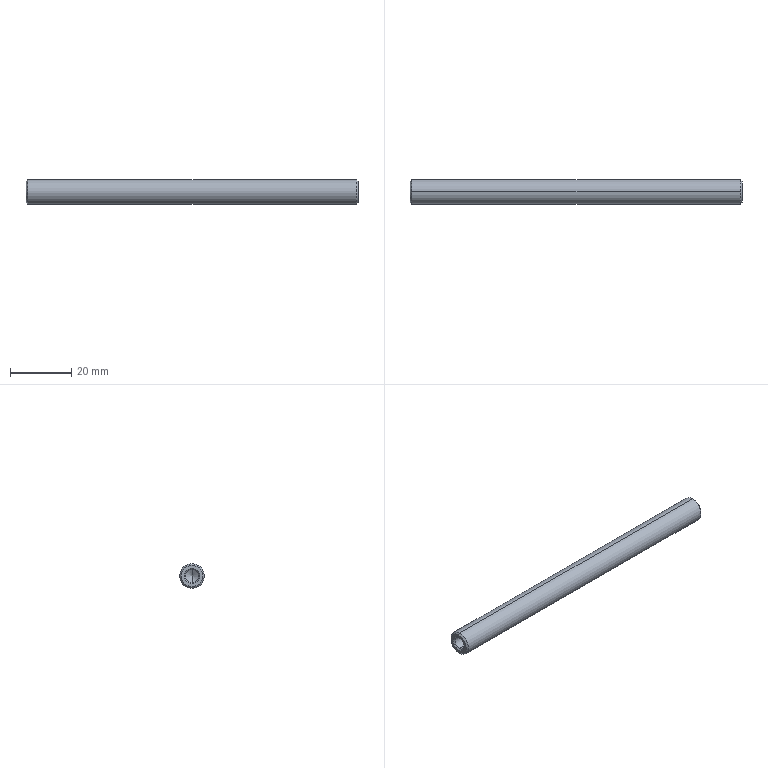Component | SolidWorks | Z-AxisSpringGuidePost-1 | 1 solid | 20 faces | box 108 x 8 x 8 mm | volume 5065 mm3 | cone 12 | cylinder 6 | plane 2 | commonest cylinder face diameters 4.2 x4 8 x2
build123d program:
from build123d import *

# Parameters (mm, degrees)
SKETCH1_R                   = 4
BOSS_EXTRUDE1_DEPTH         = 108
CHAMFER1_SIZE               = 0.5
M5_TAPPED_HOLE1_D           = 4.2
M5_TAPPED_HOLE1_DEPTH       = 12.4
M5_TAPPED_HOLE1_CSINK_D     = 5.05
M5_TAPPED_HOLE1_CSINK_ANGLE = 90
M5_TAPPED_HOLE1_TIP         = 1.262
M5_TAPPED_HOLE2_D           = 4.2
M5_TAPPED_HOLE2_DEPTH       = 12.4
M5_TAPPED_HOLE2_CSINK_D     = 5.05
M5_TAPPED_HOLE2_CSINK_ANGLE = 90
M5_TAPPED_HOLE2_TIP         = 1.262


with BuildPart() as part:
    # Sketch1 → Boss-Extrude1 (new body)
    with BuildSketch(Plane.XY):
        Circle(SKETCH1_R)
    extrude(amount=BOSS_EXTRUDE1_DEPTH)

    # Chamfer1
    chamfer1_edges = [part.edges().sort_by_distance(p)[0] for p in [
        (-4, 0, 0),
        (-4, 0, 108),
    ]]
    chamfer(chamfer1_edges, length=CHAMFER1_SIZE)

    # M5 Tapped Hole1
    with Locations(Plane(origin=(0, 0, 0), x_dir=(-1, 0, 0), z_dir=(0, 0, -1))):
        with Locations((0, 0)):
            CounterSinkHole(M5_TAPPED_HOLE1_D / 2, M5_TAPPED_HOLE1_CSINK_D / 2, depth=M5_TAPPED_HOLE1_DEPTH, counter_sink_angle=M5_TAPPED_HOLE1_CSINK_ANGLE)
            with Locations((0, 0, -(M5_TAPPED_HOLE1_DEPTH + M5_TAPPED_HOLE1_TIP / 2))):  # 118° drill point
                Cone(0, M5_TAPPED_HOLE1_D / 2, M5_TAPPED_HOLE1_TIP, mode=Mode.SUBTRACT)

    # M5 Tapped Hole2
    with Locations(Plane.XY.offset(108)):
        with Locations((0, 0)):
            CounterSinkHole(M5_TAPPED_HOLE2_D / 2, M5_TAPPED_HOLE2_CSINK_D / 2, depth=M5_TAPPED_HOLE2_DEPTH, counter_sink_angle=M5_TAPPED_HOLE2_CSINK_ANGLE)
            with Locations((0, 0, -(M5_TAPPED_HOLE2_DEPTH + M5_TAPPED_HOLE2_TIP / 2))):  # 118° drill point
                Cone(0, M5_TAPPED_HOLE2_D / 2, M5_TAPPED_HOLE2_TIP, mode=Mode.SUBTRACT)


solid = part.part

# Placed as in the assembly
solid = solid.moved(Location((-78.981, 68.516, 82), (0, 90, 0)))